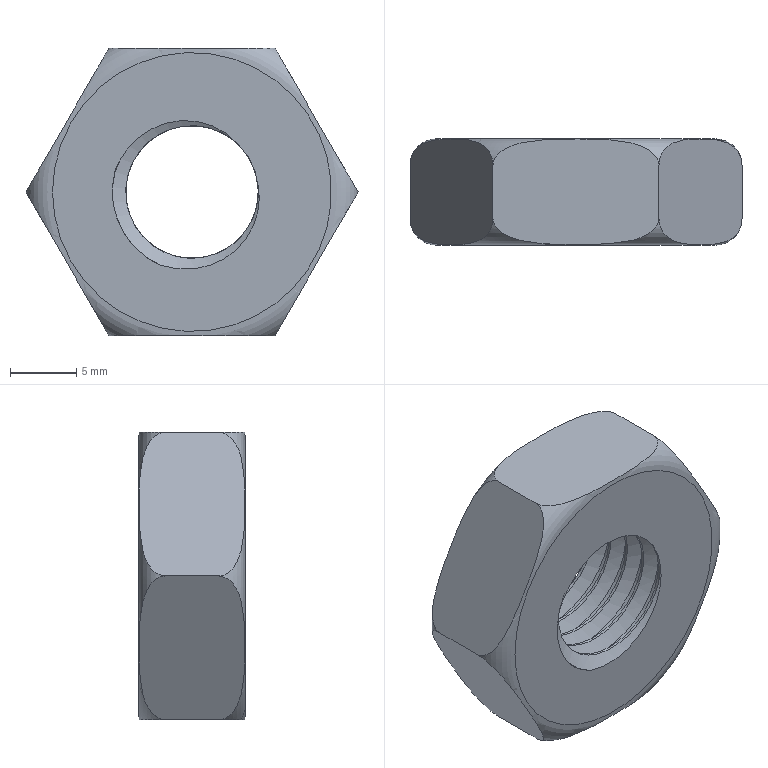Component | NX | JJZ-006 | 1 solid | 14 faces | volume 2451 mm3 | plane 8 | torus 2 | cylinder 2 | spline 2 | commonest cylinder face diameters 10 x1 12 x1